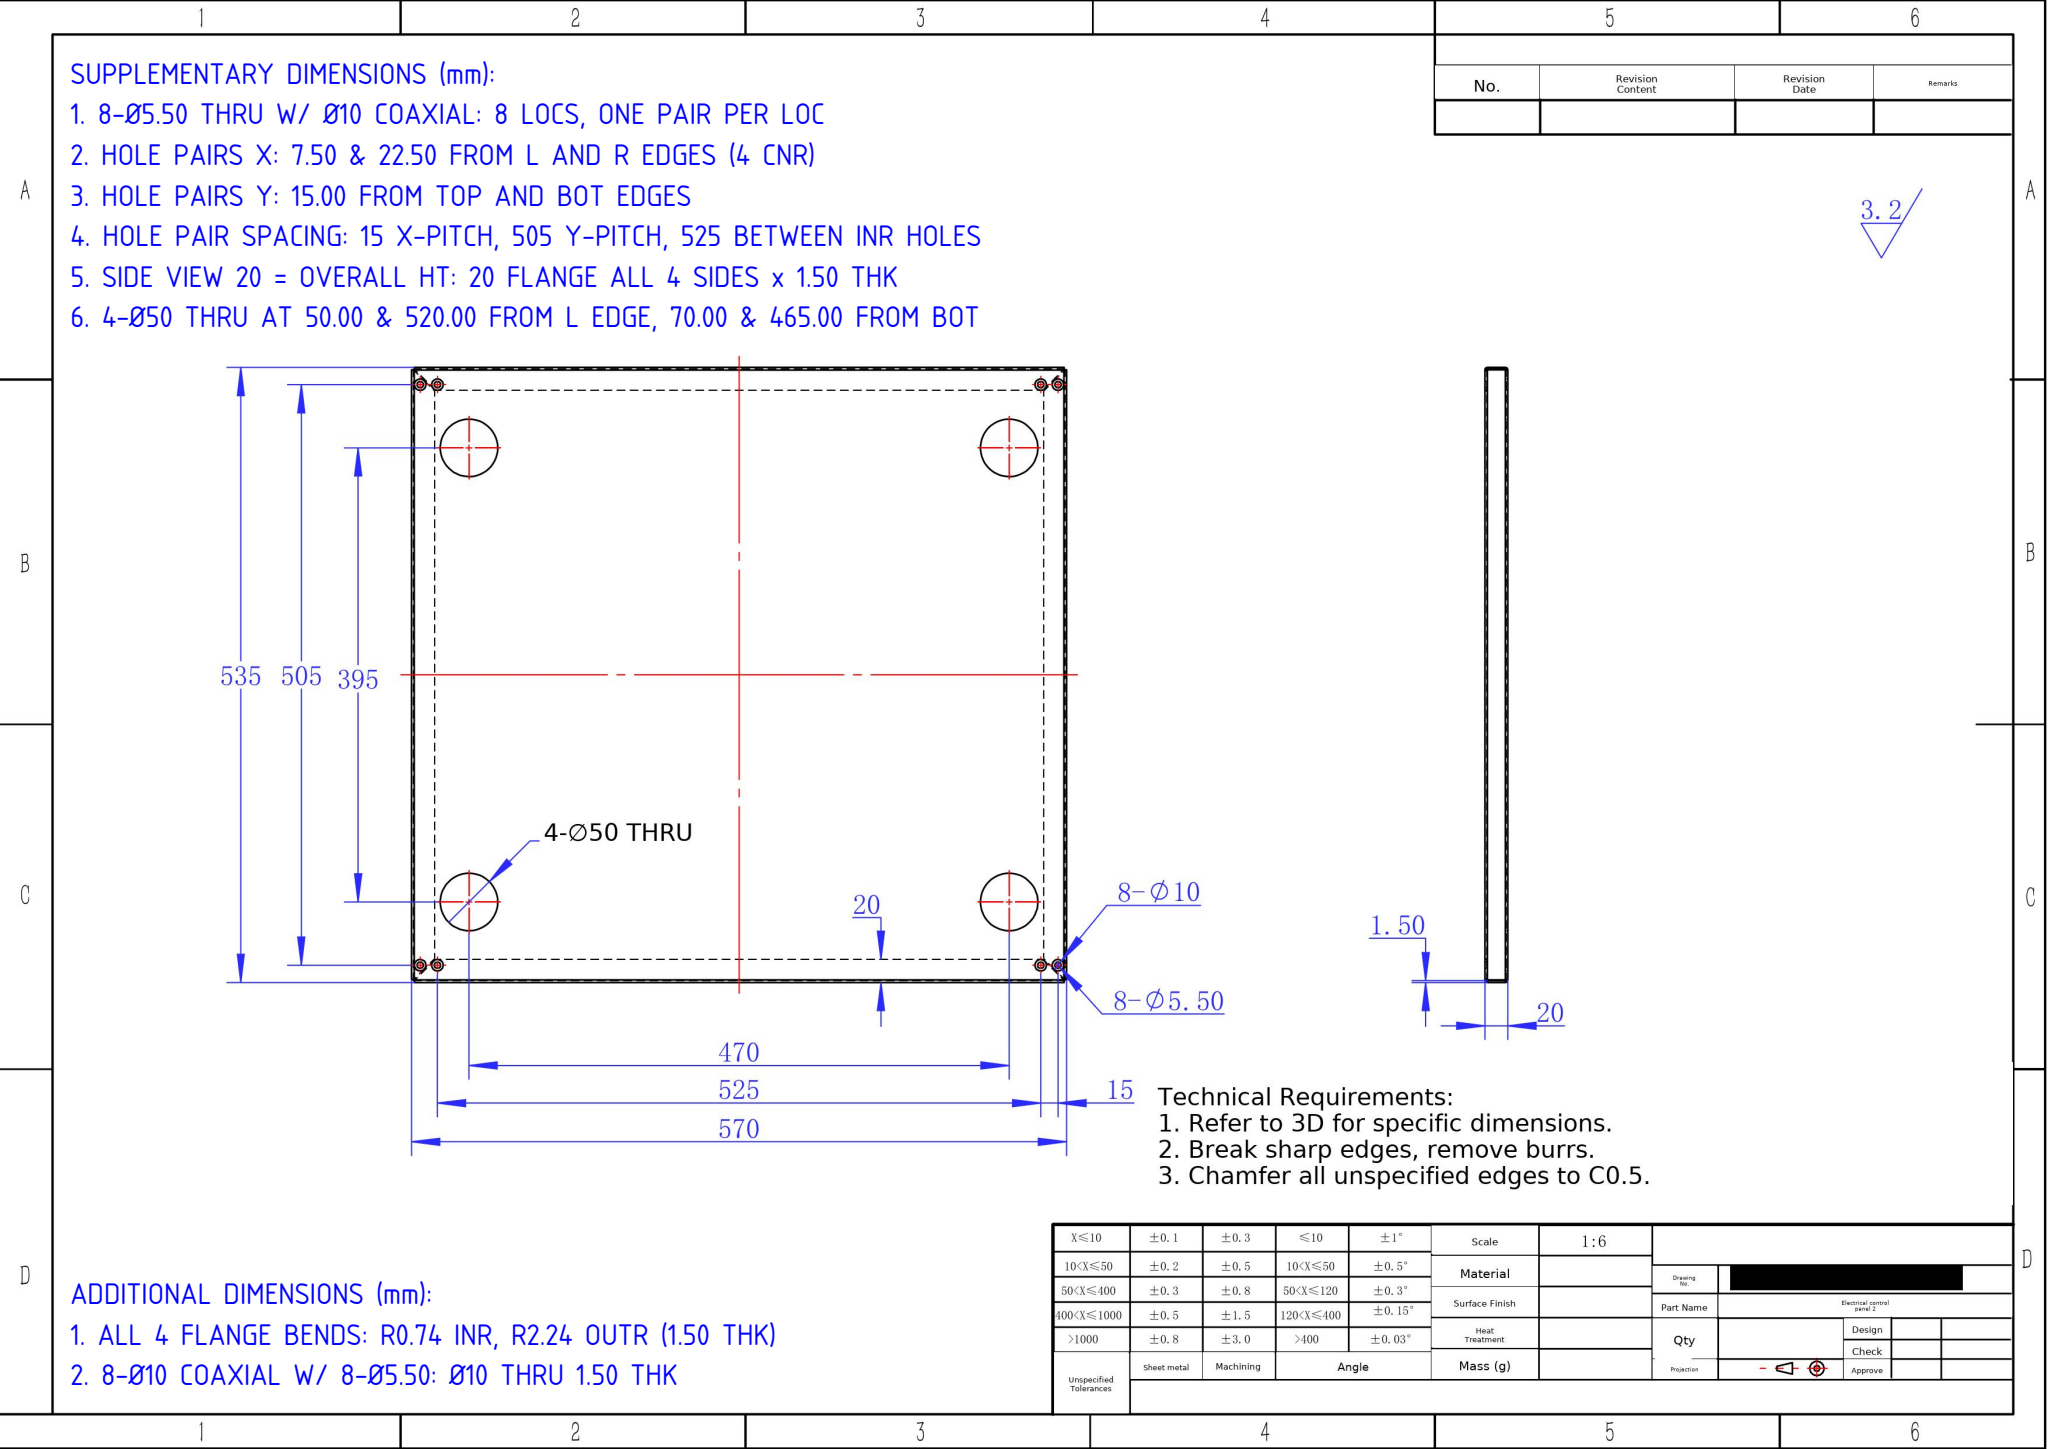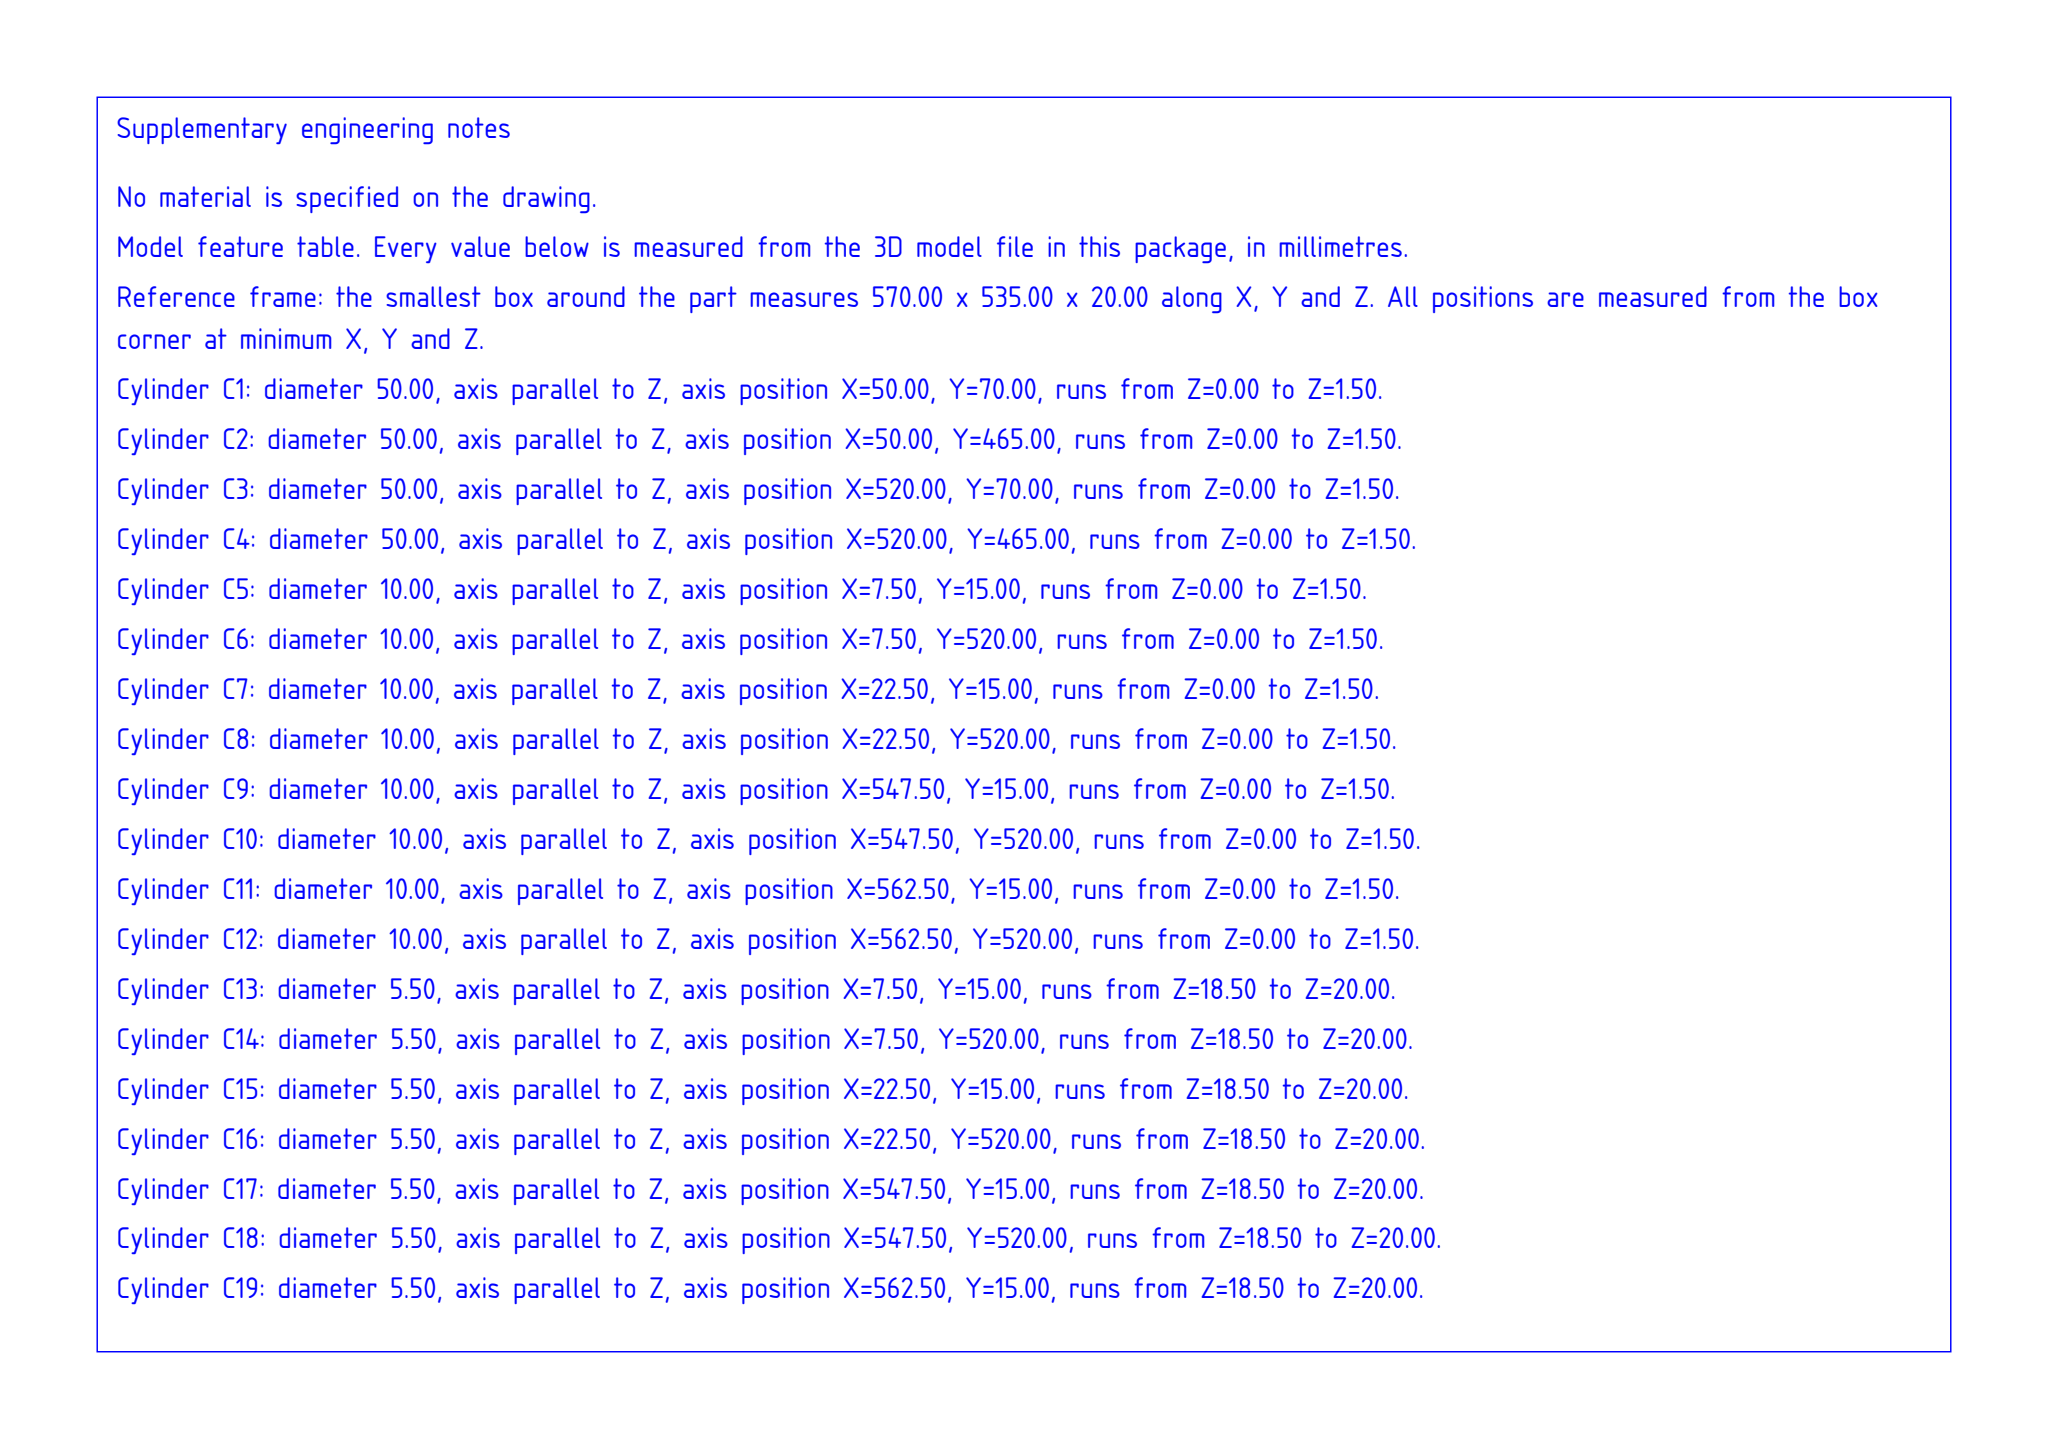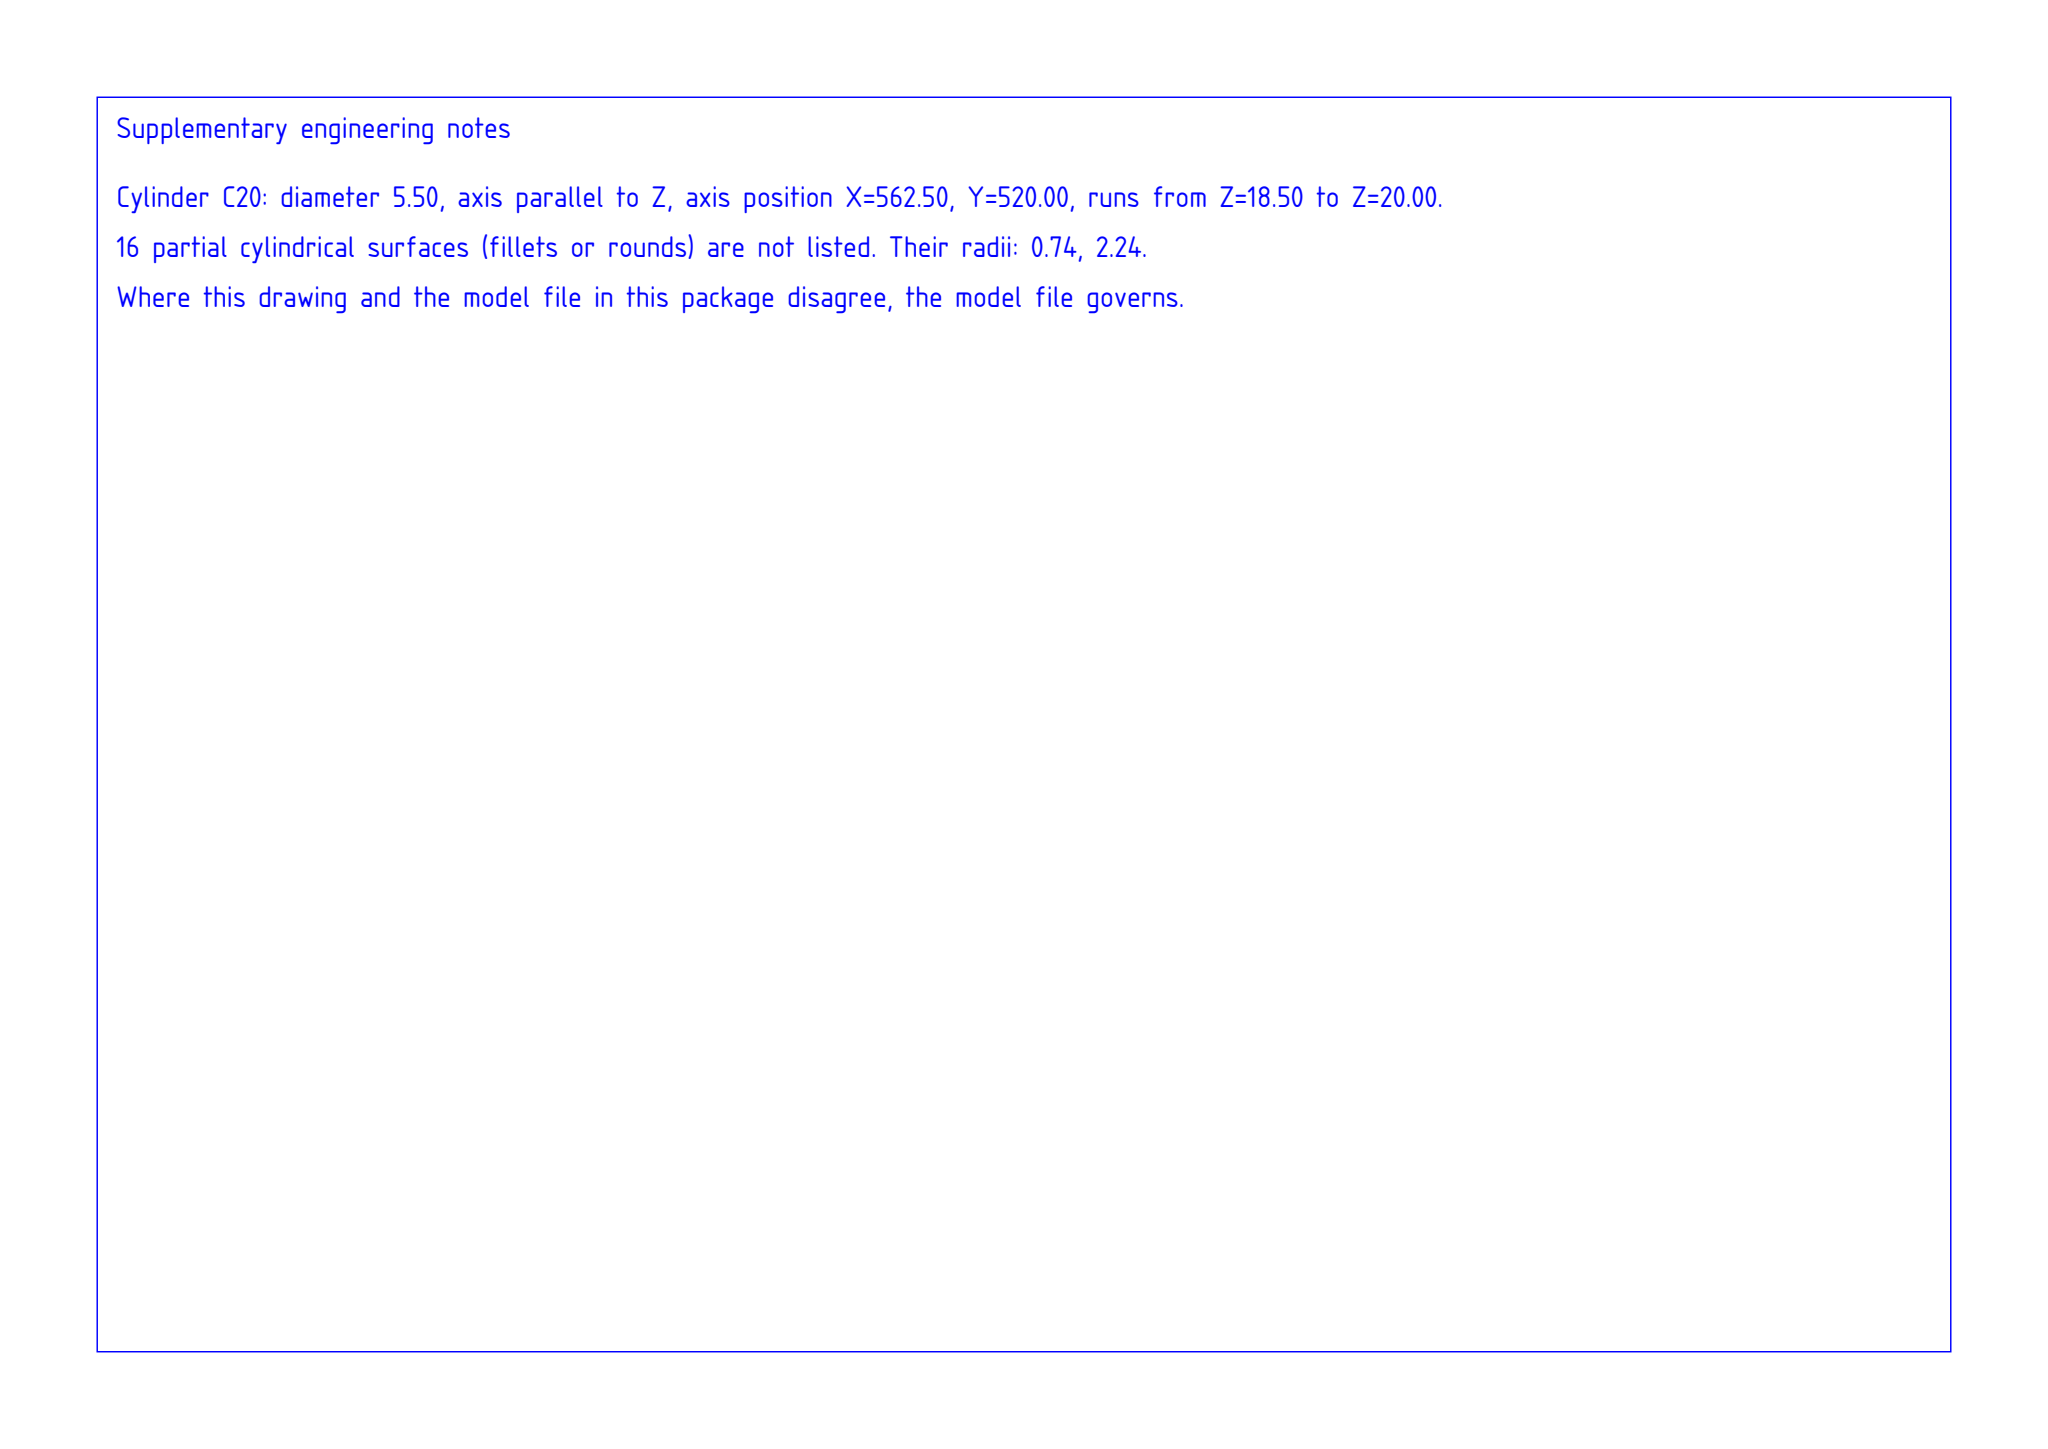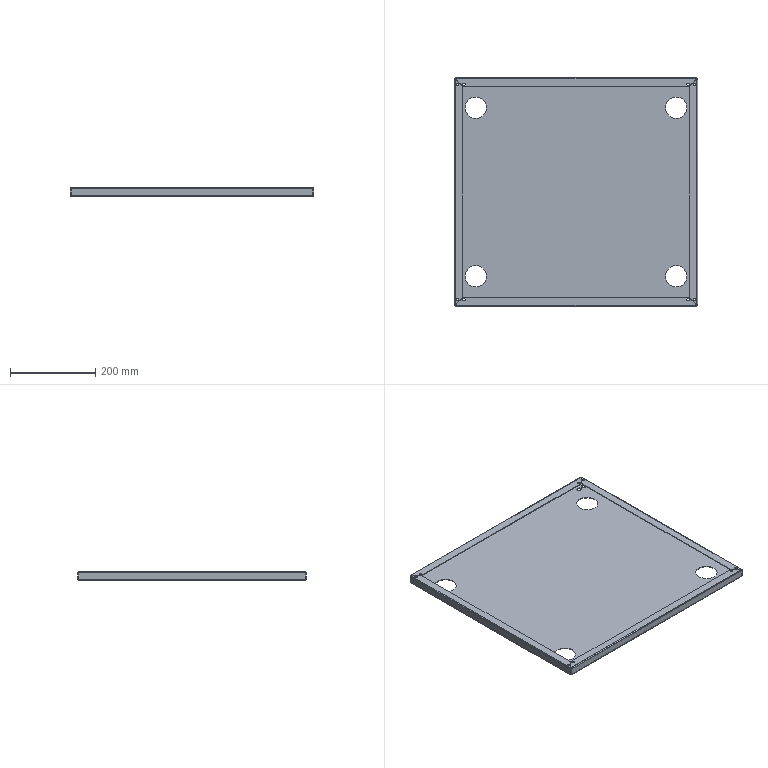Part | SolidWorks | mm | 1 solid | 110 faces | box 570 x 535 x 20 mm | volume 559805 mm3 | cylinder 56 | plane 38 | spline 16 | commonest cylinder face diameters 10 x16 5.5 x16 50 x8 4.473 x8 1.473 x8